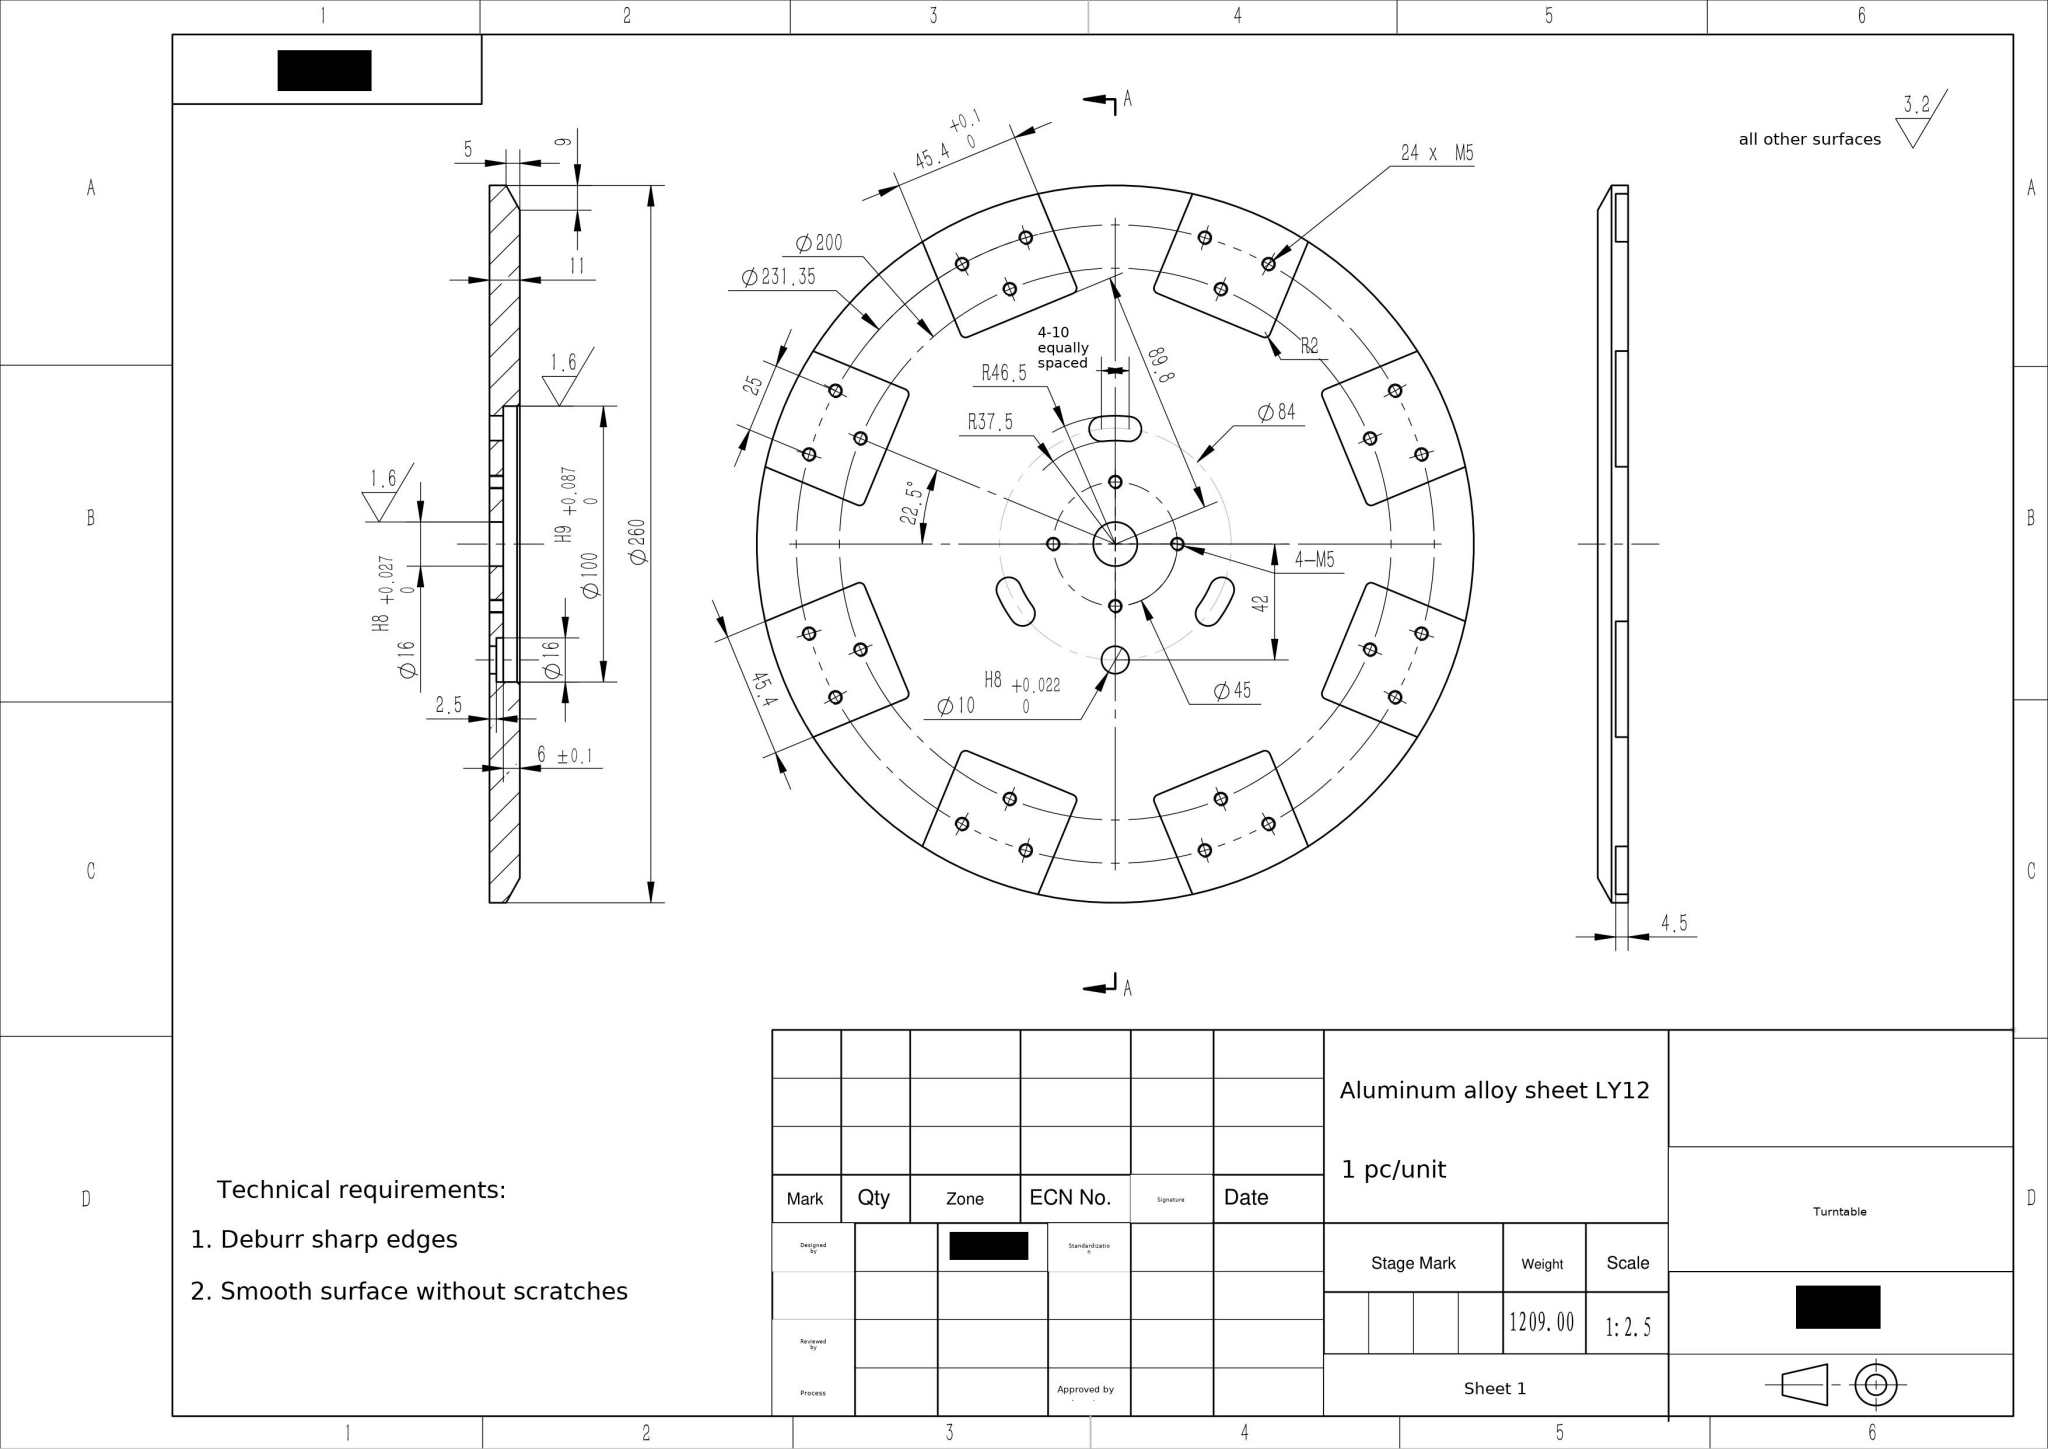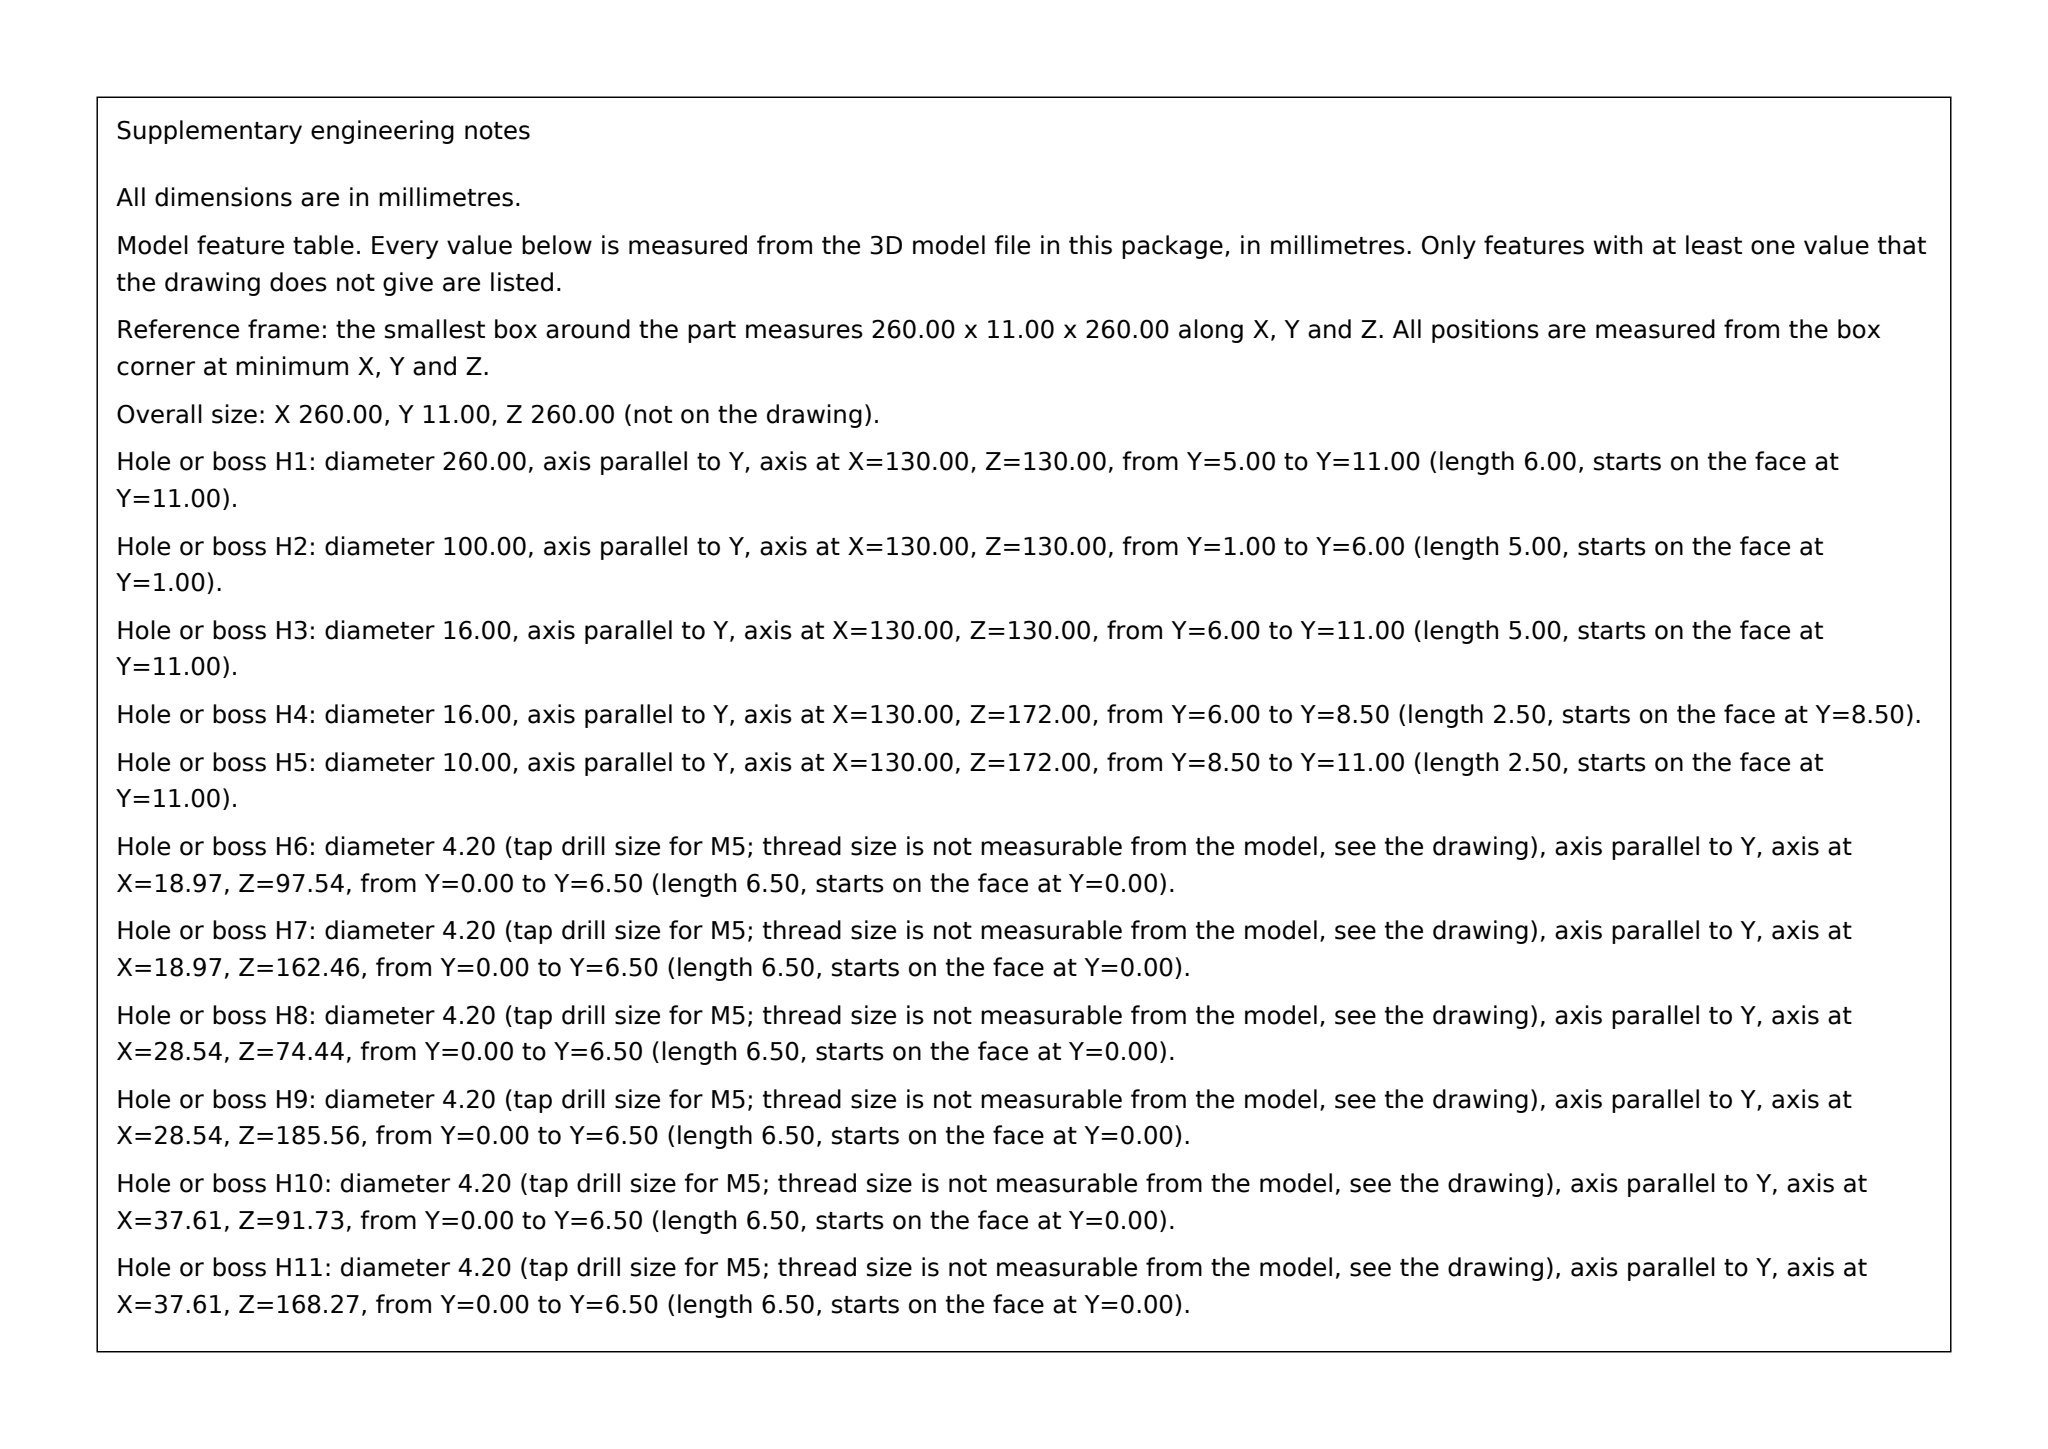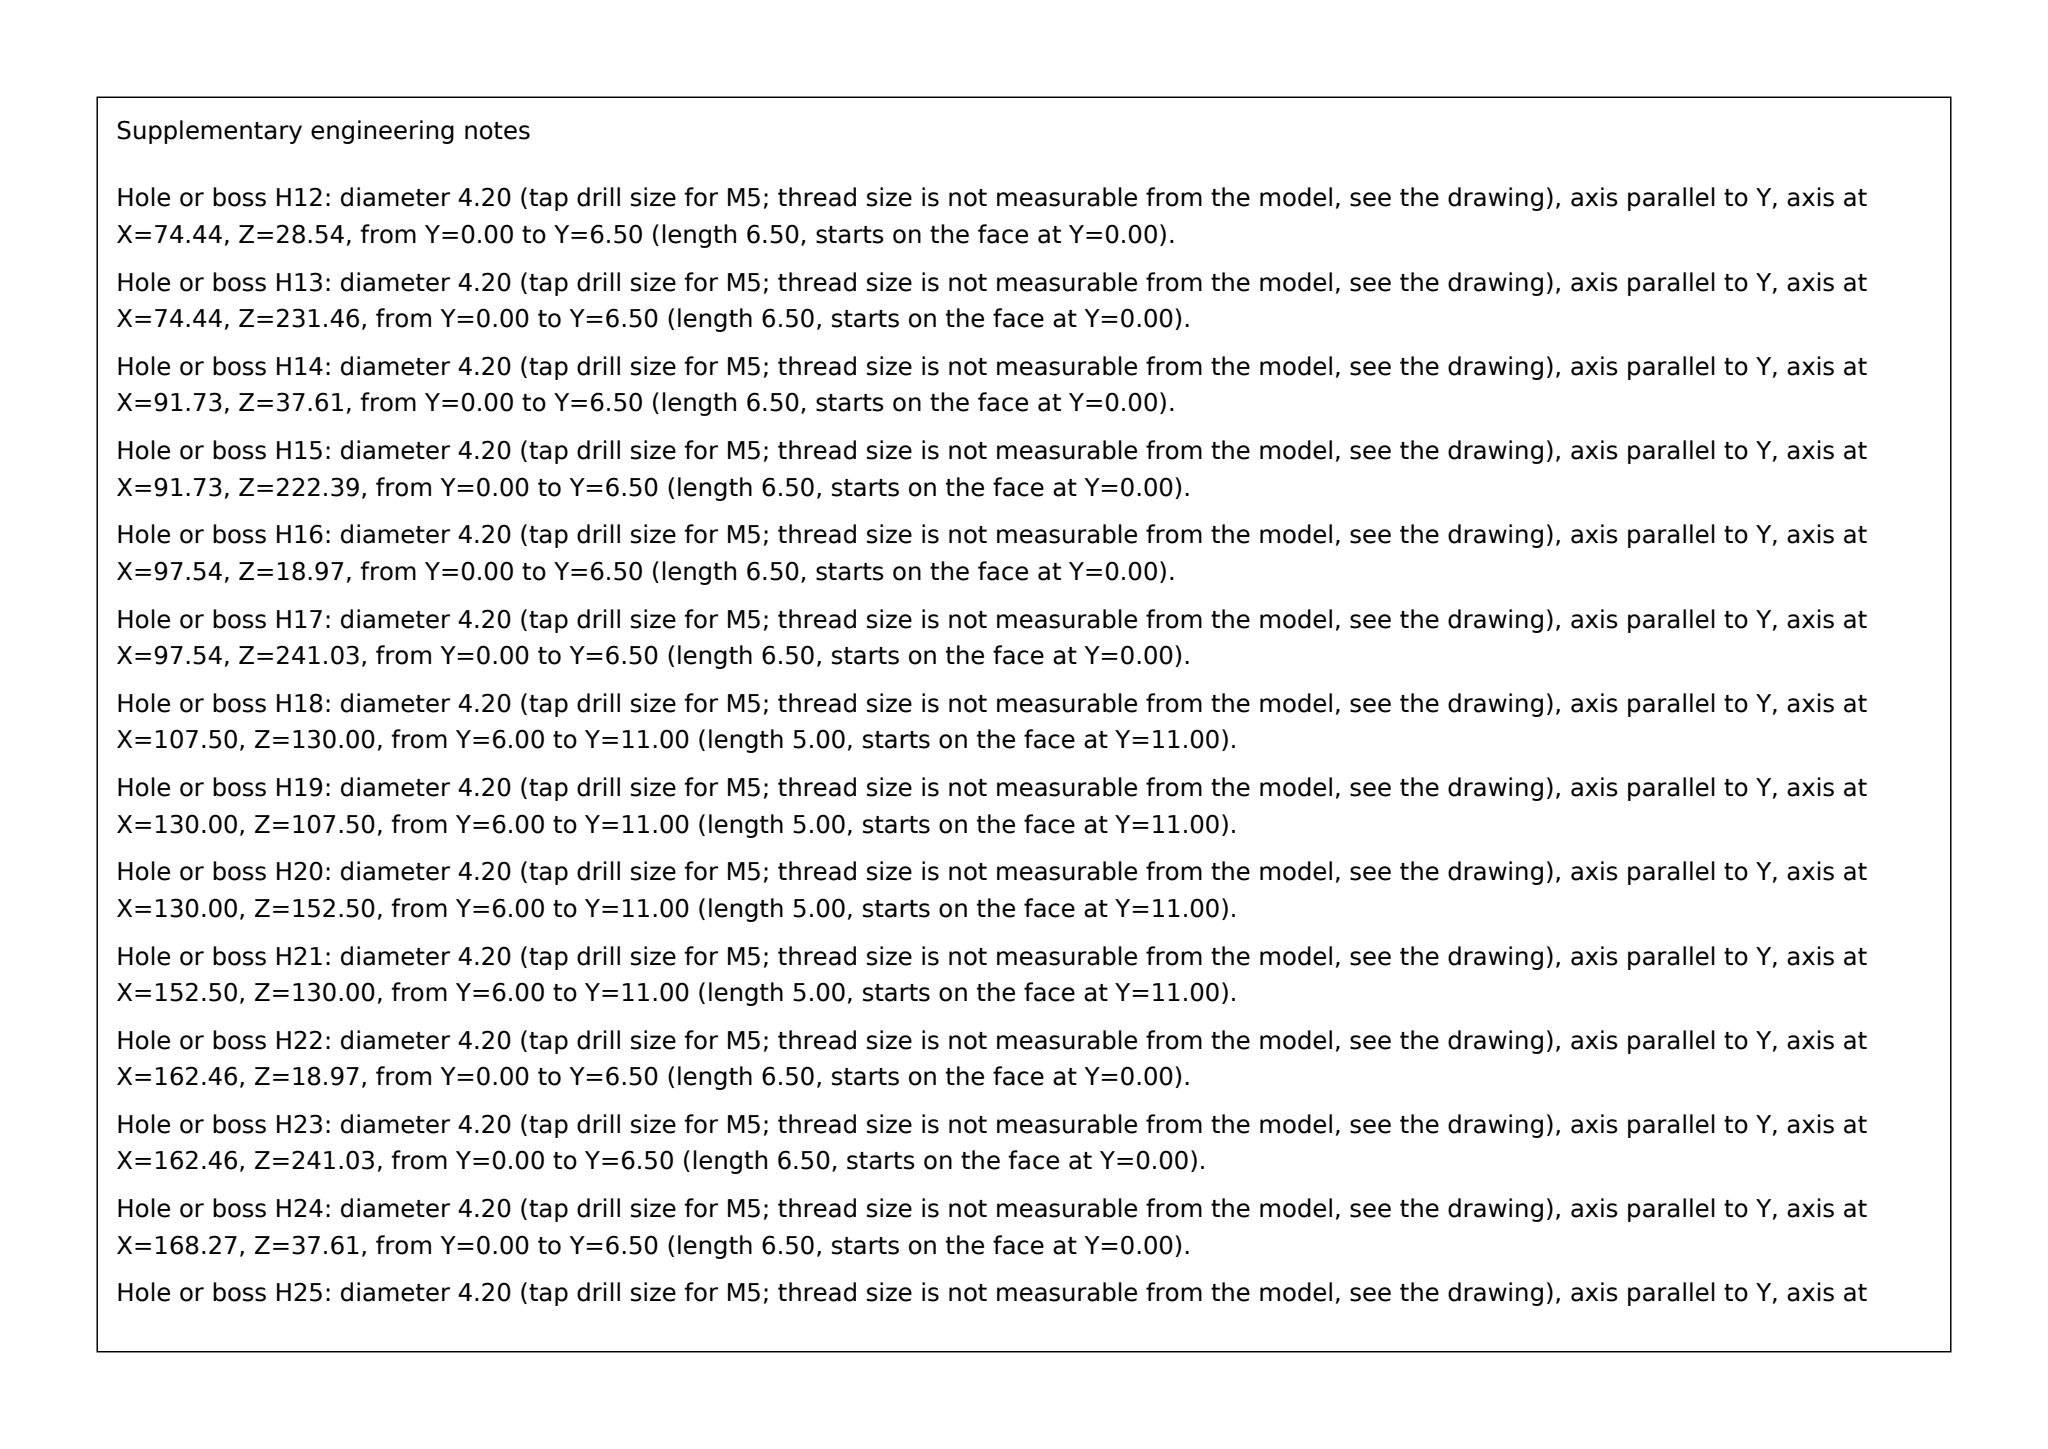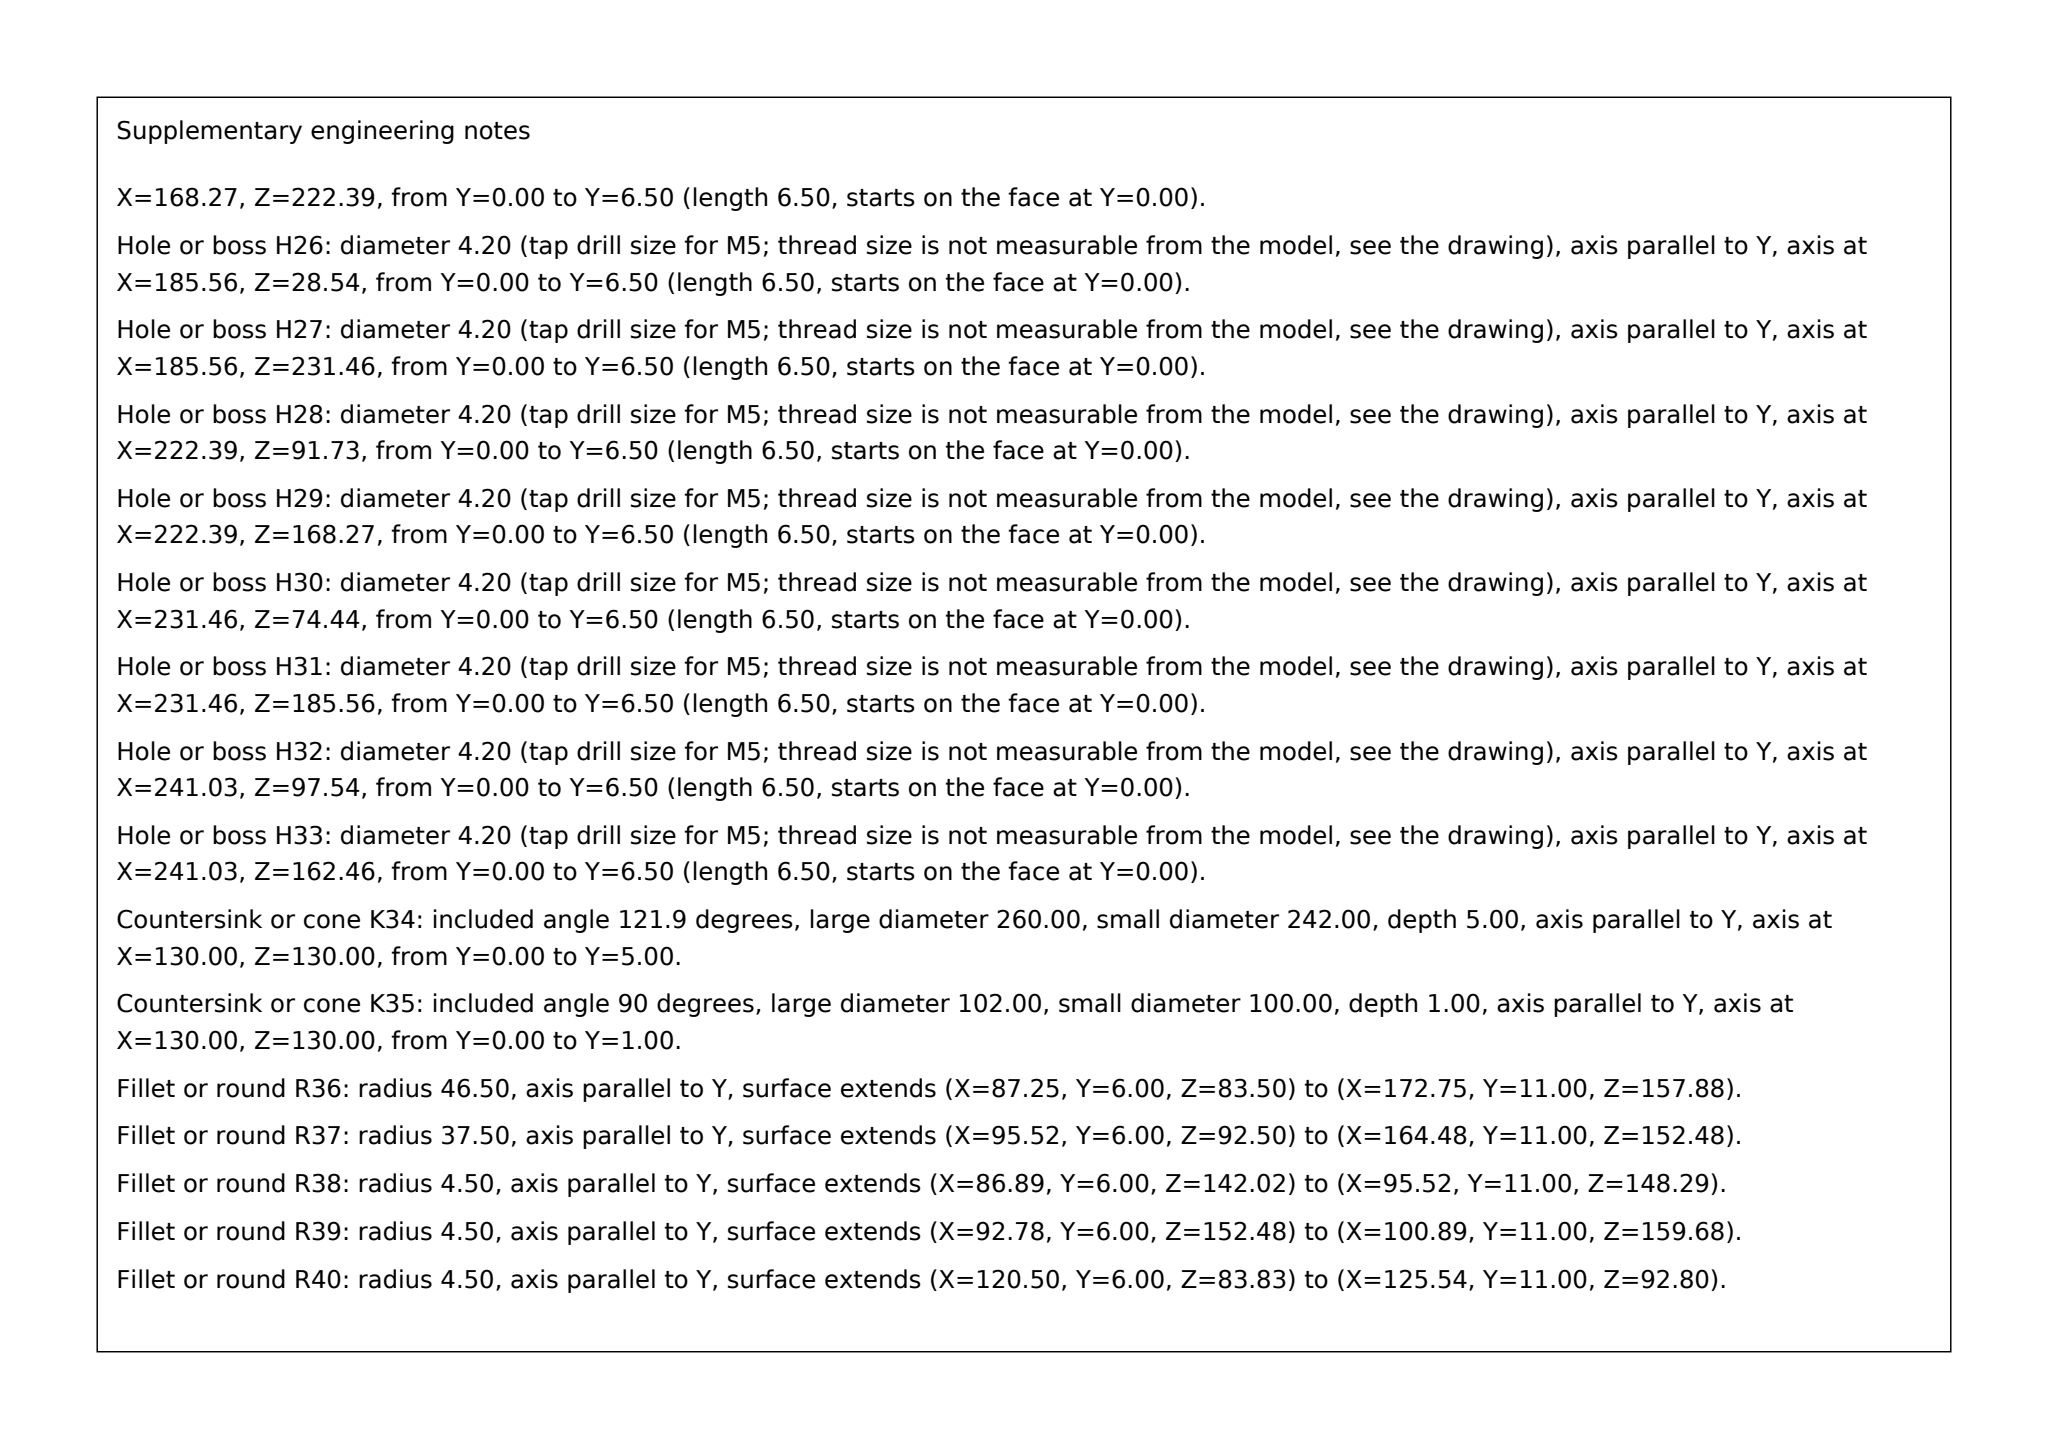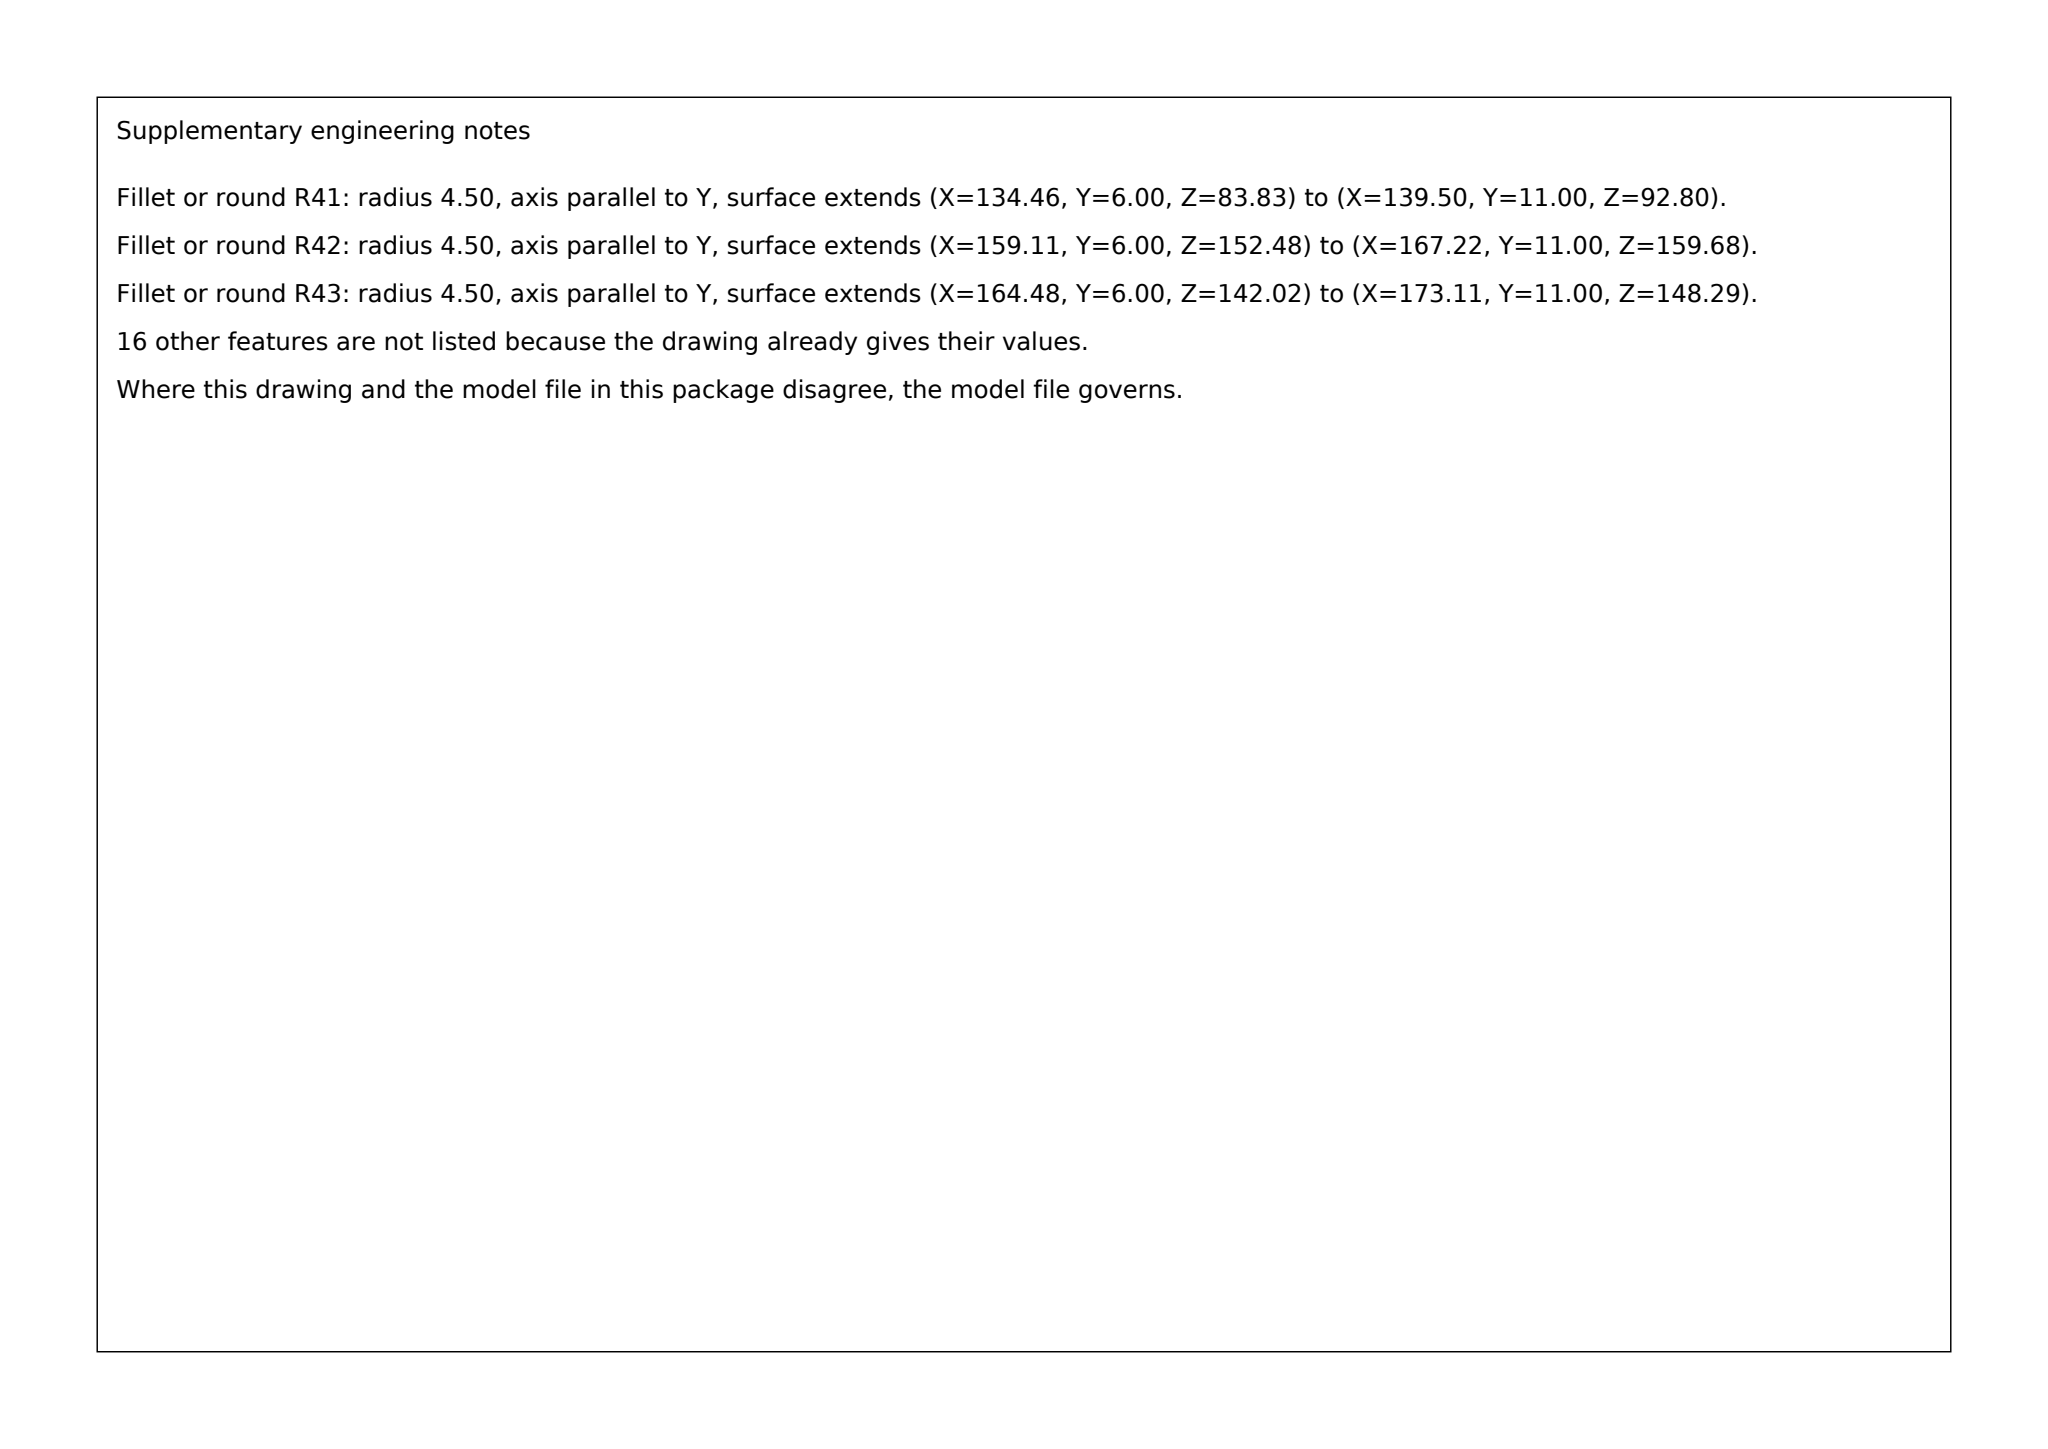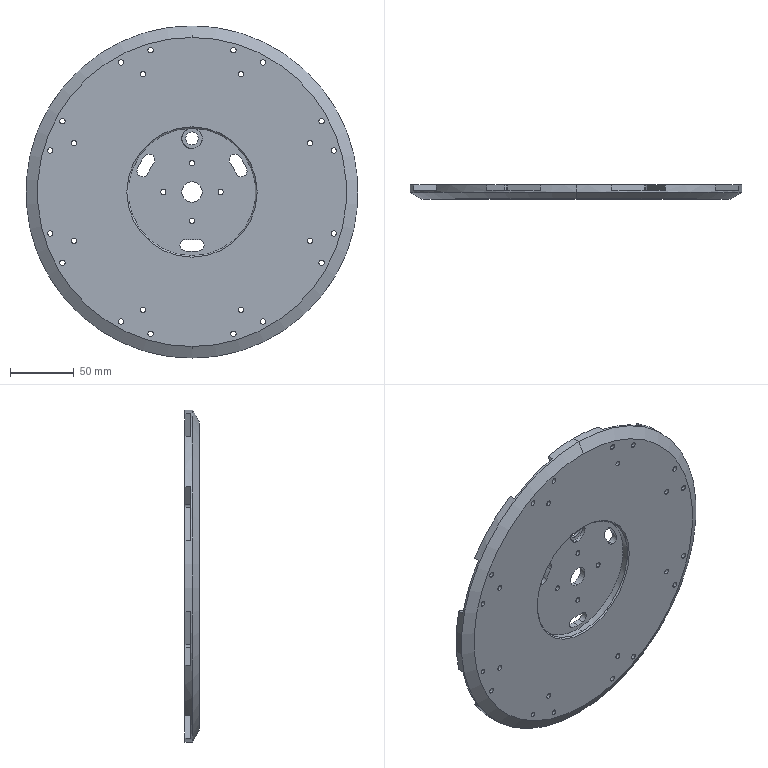Part | SolidWorks | mm | material Aluminum alloy sheet LY12 | 1 solid | 142 faces | box 260 x 11 x 260 mm | volume 447779 mm3 | cylinder 102 | plane 36 | cone 4 | commonest cylinder face diameters 4.2 x56 4 x20 9 x8 16 x4 75 x4 93 x4 100 x2 260 x2
build123d program:
from build123d import *

# Parameters (mm, degrees)
SKETCH1_R                  = 130
BOSS_EXTRUDE1_DEPTH        = 11
CUT_EXTRUDE1_DEPTH         = 4.5
M5_TAPPED_HOLE1_D          = 4.2
FILLET1_R                  = 2
CIRPATTERN1_COUNT          = 8
FILLET1_OF_CIRPATTERN1_R   = 2
SKETCH5_R                  = 50
CUT_EXTRUDE2_DEPTH         = 6
CUT_EXTRUDE3_DEPTH         = 184.946
CIRPATTERN2_COUNT          = 3
SKETCH10_R                 = 5
CUT_EXTRUDE4_DEPTH         = 184.946
CHAMFER1_SIZE              = 9
CHAMFER1_SIZE2             = 5
M5_TAPPED_HOLE2_D          = 4.2
F_20_0_20_DIAMETER_HOLE1_D = 16
CIRPATTERN3_COUNT          = 4
CHAMFER2_SIZE              = 1
SKETCH16_R                 = 8
CUT_EXTRUDE5_DEPTH         = 2.5


with BuildPart() as part:
    # Sketch1 → Boss-Extrude1 (new body)
    with BuildSketch(Plane(origin=(0, 0, 0), x_dir=(1, 0, 0), z_dir=(0, 1, 0))):
        with Locations(Location((0, 0, 0), (0, 0, 270))):
            Circle(SKETCH1_R)
    extrude(amount=BOSS_EXTRUDE1_DEPTH)

    # Sketch2 → Cut-Extrude1 (cut)
    with BuildSketch(Plane(origin=(0, 11, 0), x_dir=(1, 0, 0), z_dir=(0, 1, 0))):
        Polygon((-55.337, -74.277), (-13.393, -91.651), (-30.69, -133.411), (-72.634, -116.037), align=None)
    cut_extrude1 = extrude(amount=-CUT_EXTRUDE1_DEPTH, mode=Mode.SUBTRACT)

    # M5 Tapped Hole1 (through all)
    with Locations(Plane(origin=(0, 6.5, 0), x_dir=(1, 0, 0), z_dir=(0, 1, 0))):
        with Locations((-38.268, -92.388), (-55.557, -101.463), (-32.46, -111.03)):
            m5_tapped_hole1 = Hole(M5_TAPPED_HOLE1_D / 2)

    # Fillet1
    fillet1_edges = [part.edges().sort_by_distance(p)[0] for p in [
        (-13.393, 8.75, 91.651),
        (-55.337, 8.75, 74.277),
    ]]
    fillet(fillet1_edges, radius=FILLET1_R)

    # CirPattern1: Cut-Extrude1, M5 Tapped Hole1 ×8 about axis
    cirpattern1_axis = Axis((0, 0, 0), (0, 1, 0))
    add([cut_extrude1.rotate(cirpattern1_axis, i * 360 / CIRPATTERN1_COUNT) for i in range(1, CIRPATTERN1_COUNT)], mode=Mode.SUBTRACT)
    add([m5_tapped_hole1.rotate(cirpattern1_axis, i * 360 / CIRPATTERN1_COUNT) for i in range(1, CIRPATTERN1_COUNT)], mode=Mode.SUBTRACT)

    # Fillet1 of CirPattern1
    fillet1_of_cirpattern1_edges = [part.edges().sort_by_distance(p)[0] for p in [
        (55.337, 8.75, 74.277),
        (13.393, 8.75, 91.651),
        (91.651, 8.75, 13.393),
        (74.277, 8.75, 55.337),
        (74.277, 8.75, -55.337),
        (91.651, 8.75, -13.393),
        (13.393, 8.75, -91.651),
        (55.337, 8.75, -74.277),
        (-55.337, 8.75, -74.277),
        (-13.393, 8.75, -91.651),
        (-91.651, 8.75, -13.393),
        (-74.277, 8.75, -55.337),
        (-74.277, 8.75, 55.337),
        (-91.651, 8.75, 13.393),
    ]]
    fillet(fillet1_of_cirpattern1_edges, radius=FILLET1_OF_CIRPATTERN1_R)

    # Sketch5 → Cut-Extrude2 (cut)
    with BuildSketch(Plane.XZ):
        with Locations(Location((0, 0, 0), (0, 0, 270))):
            Circle(SKETCH5_R)
    extrude(amount=-CUT_EXTRUDE2_DEPTH, mode=Mode.SUBTRACT)

    # Sketch9 → Cut-Extrude3 (cut, through all)
    with BuildSketch(Plane(origin=(0, 6, 0), x_dir=(1, 0, 0), z_dir=(0, 1, 0))):
        with BuildLine():
            ThreePointArc((5.536, 46.169), (0, 46.5), (-5.536, 46.169))
            ThreePointArc((-5.536, 46.169), (-9.468, 41.166), (-4.464, 37.233))
            ThreePointArc((-4.464, 37.233), (0, 37.5), (4.464, 37.233))
            ThreePointArc((4.464, 37.233), (9.468, 41.166), (5.536, 46.169))
        make_face()
    cut_extrude3 = extrude(amount=CUT_EXTRUDE3_DEPTH, mode=Mode.SUBTRACT)

    # CirPattern2: Cut-Extrude3 ×3 about axis
    cirpattern2_axis = Axis((0, 0, 0), (0, 1, 0))
    for i in range(1, CIRPATTERN2_COUNT):
        add(cut_extrude3.rotate(cirpattern2_axis, i * 360 / CIRPATTERN2_COUNT), mode=Mode.SUBTRACT)

    # Sketch10 → Cut-Extrude4 (cut, through all)
    with BuildSketch(Plane.XZ.offset(-6)):
        with Locations(Location((0, 42, 0), (0, 0, 270))):
            Circle(SKETCH10_R)
    extrude(amount=-CUT_EXTRUDE4_DEPTH, mode=Mode.SUBTRACT)

    # Chamfer1
    chamfer1_edges = [part.edges().sort_by_distance(p)[0] for p in [
        (0, 0, -130),
    ]]
    chamfer1_side = [part.faces().sort_by_distance(p)[0] for p in [
        (0, 0, -126.323),
    ]]
    chamfer(chamfer1_edges, length=CHAMFER1_SIZE, length2=CHAMFER1_SIZE2, reference=chamfer1_side[0])

    # M5 Tapped Hole2 (through all)
    with Locations(Plane(origin=(0, 11, 0), x_dir=(1, 0, 0), z_dir=(0, 1, 0))):
        with Locations((-22.5, 0)):
            m5_tapped_hole2 = Hole(M5_TAPPED_HOLE2_D / 2)

    # 20.0 _20_ Diameter Hole1 (through all)
    with Locations(Plane(origin=(0, 11, 0), x_dir=(1, 0, 0), z_dir=(0, 1, 0))):
        with Locations((0, 0)):
            Hole(F_20_0_20_DIAMETER_HOLE1_D / 2)

    # CirPattern3: M5 Tapped Hole2 ×4 about axis
    cirpattern3_axis = Axis((0, 0, 0), (0, 1, 0))
    for i in range(1, CIRPATTERN3_COUNT):
        add(m5_tapped_hole2.rotate(cirpattern3_axis, i * 360 / CIRPATTERN3_COUNT), mode=Mode.SUBTRACT)

    # Chamfer2
    chamfer2_edges = [part.edges().sort_by_distance(p)[0] for p in [
        (0, 0, 50),
    ]]
    chamfer(chamfer2_edges, length=CHAMFER2_SIZE)

    # Sketch16 → Cut-Extrude5 (cut)
    with BuildSketch(Plane.XZ.offset(-6)):
        with Locations(Location((0, 42, 0), (0, 0, 270))):
            Circle(SKETCH16_R)
    extrude(amount=-CUT_EXTRUDE5_DEPTH, mode=Mode.SUBTRACT)


solid = part.part